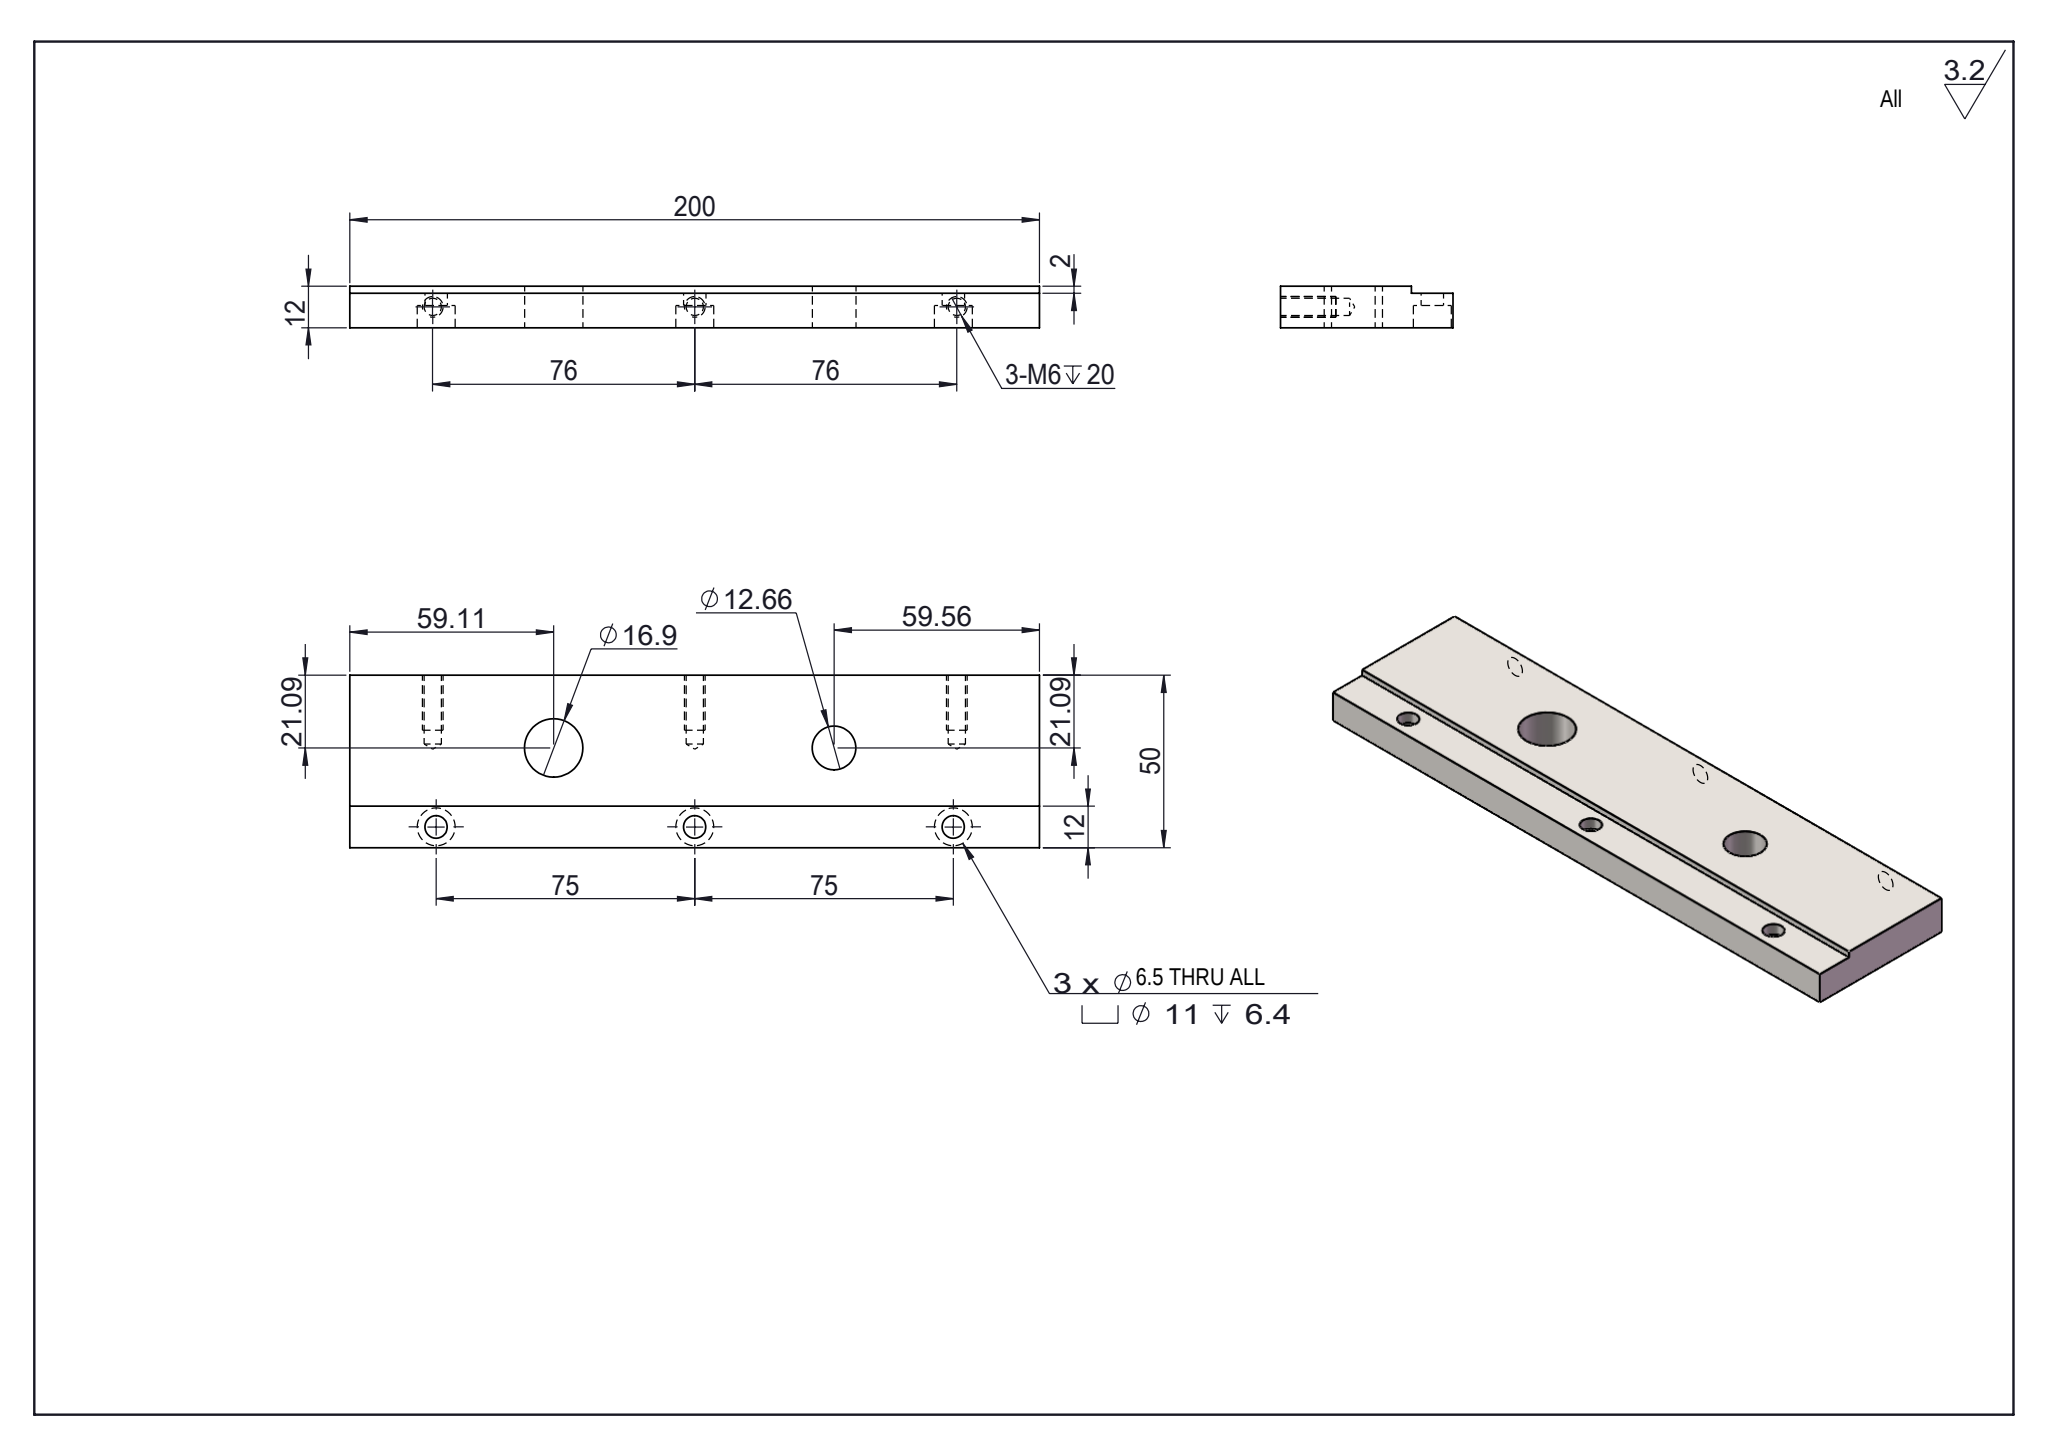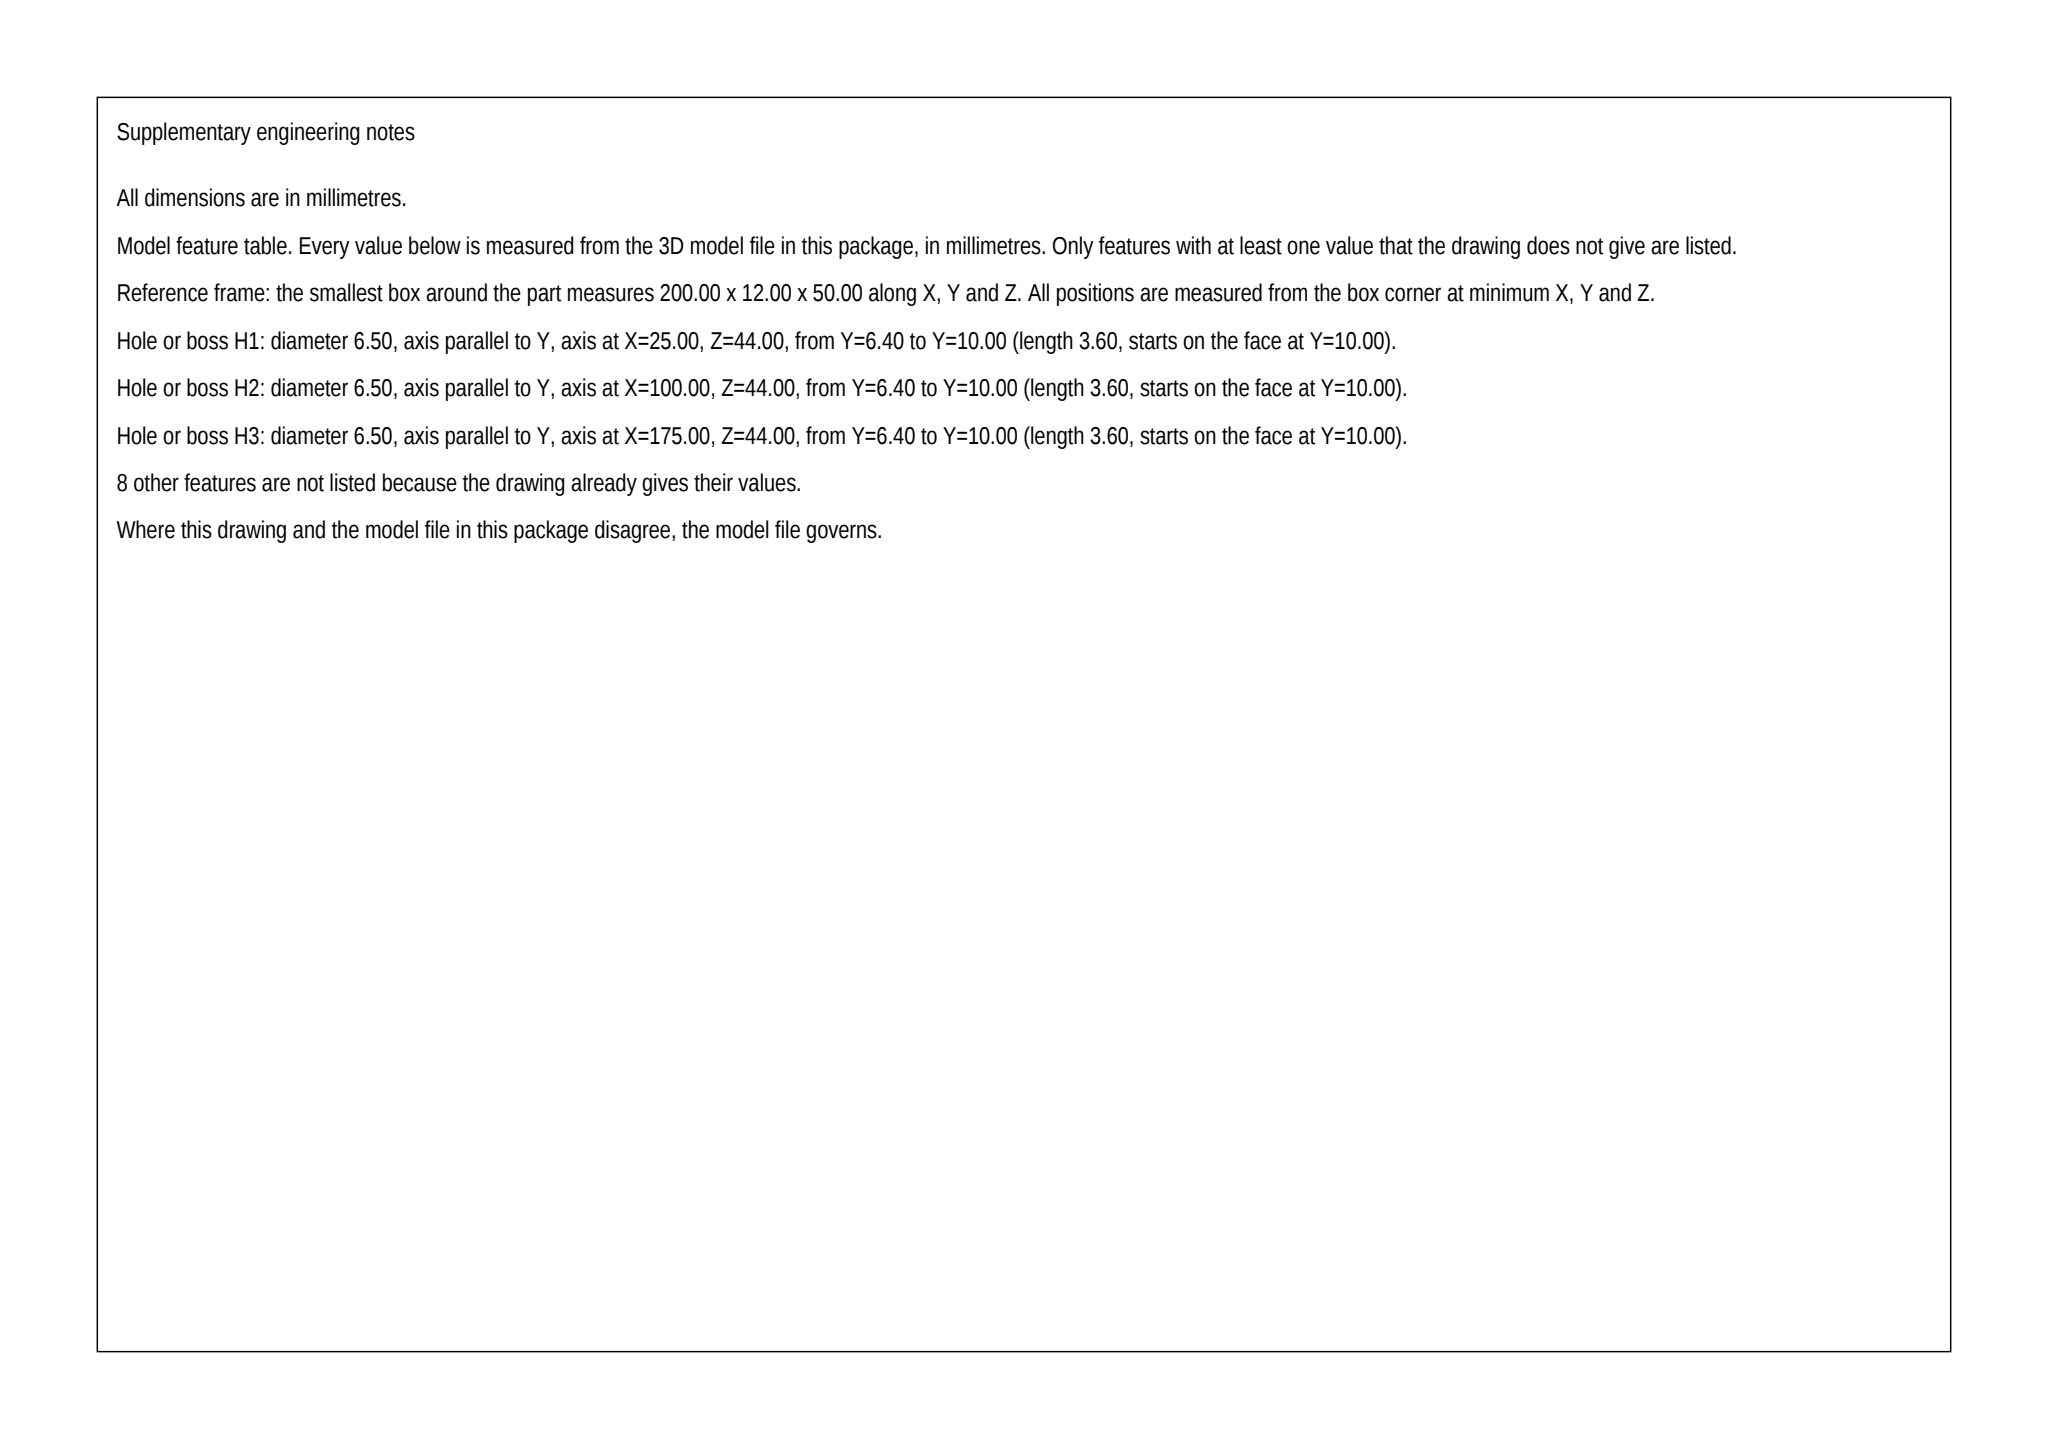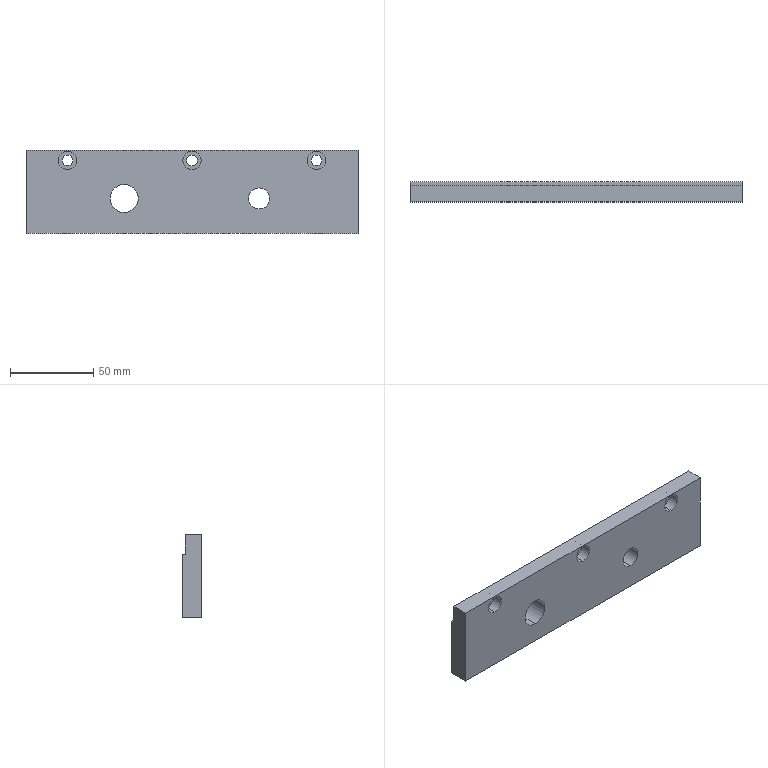Part | SolidWorks | mm | 1 solid | 39 faces | box 200 x 12 x 50 mm | volume 107607 mm3 | cylinder 22 | plane 11 | cone 6 | commonest cylinder face diameters 11 x6 6.5 x6 5 x6 16.903 x2 12.657 x2
build123d program:
from build123d import *

# Parameters (mm, degrees)
SKETCH1_W                                           = 200
SKETCH1_H                                           = 12
BOSS_EXTRUDE1_DEPTH                                 = 50
M6_TAPPED_HOLE1_D                                   = 5
M6_TAPPED_HOLE1_DEPTH                               = 20
M6_TAPPED_HOLE1_TIP                                 = 1.502
SKETCH4_W                                           = 200
SKETCH4_H                                           = 12
CUT_EXTRUDE1_DEPTH                                  = 2
CYLINDRICAL_COUNTERSUNK_HOLE_FOR_M6_HEX_D           = 6.5
CYLINDRICAL_COUNTERSUNK_HOLE_FOR_M6_HEX_CBORE_D     = 11
CYLINDRICAL_COUNTERSUNK_HOLE_FOR_M6_HEX_CBORE_DEPTH = 6.4
SKETCH7_R                                           = 8.451
SKETCH7_R_2                                         = 6.328
CUT_EXTRUDE2_DEPTH                                  = 80


with BuildPart() as part:
    # Sketch1 → Boss-Extrude1 (new body)
    with BuildSketch(Plane.XY):
        with Locations((758.704, 45.519)):
            Rectangle(SKETCH1_W, SKETCH1_H)
    extrude(amount=-BOSS_EXTRUDE1_DEPTH)

    # M6 Tapped Hole1
    with Locations(Plane(origin=(0, 0, -50), x_dir=(-1, 0, 0), z_dir=(0, 0, -1))):
        with Locations((-834.704, 45.519), (-758.704, 45.519), (-682.704, 45.519)):
            Hole(M6_TAPPED_HOLE1_D / 2, depth=M6_TAPPED_HOLE1_DEPTH)
            with Locations((0, 0, -(M6_TAPPED_HOLE1_DEPTH + M6_TAPPED_HOLE1_TIP / 2))):  # 118° drill point
                Cone(0, M6_TAPPED_HOLE1_D / 2, M6_TAPPED_HOLE1_TIP, mode=Mode.SUBTRACT)

    # Sketch4 → Cut-Extrude1 (cut)
    with BuildSketch(Plane(origin=(0, 51.519, 0), x_dir=(1, 0, 0), z_dir=(0, 1, 0))):
        with Locations((758.704, 6)):
            Rectangle(SKETCH4_W, SKETCH4_H)
    extrude(amount=-CUT_EXTRUDE1_DEPTH, mode=Mode.SUBTRACT)

    # Cylindrical Countersunk Hole for M6 Hex (through all)
    with Locations(Plane(origin=(0, 39.519, 0), x_dir=(-1, 0, 0), z_dir=(0, -1, 0))):
        with Locations((-833.704, 6), (-758.704, 6), (-683.704, 6)):
            CounterBoreHole(CYLINDRICAL_COUNTERSUNK_HOLE_FOR_M6_HEX_D / 2, CYLINDRICAL_COUNTERSUNK_HOLE_FOR_M6_HEX_CBORE_D / 2, CYLINDRICAL_COUNTERSUNK_HOLE_FOR_M6_HEX_CBORE_DEPTH)

    # Sketch7 → Cut-Extrude2 (cut)
    with BuildSketch(Plane(origin=(0, 51.519, 0), x_dir=(1, 0, 0), z_dir=(0, 1, 0))):
        with Locations(Location((717.813, 28.91, 0), (0, 0, 270))):
            Circle(SKETCH7_R)
        with Locations(Location((799.141, 28.91, 0), (0, 0, 270))):
            Circle(SKETCH7_R_2)
    extrude(amount=-CUT_EXTRUDE2_DEPTH, mode=Mode.SUBTRACT)


solid = part.part